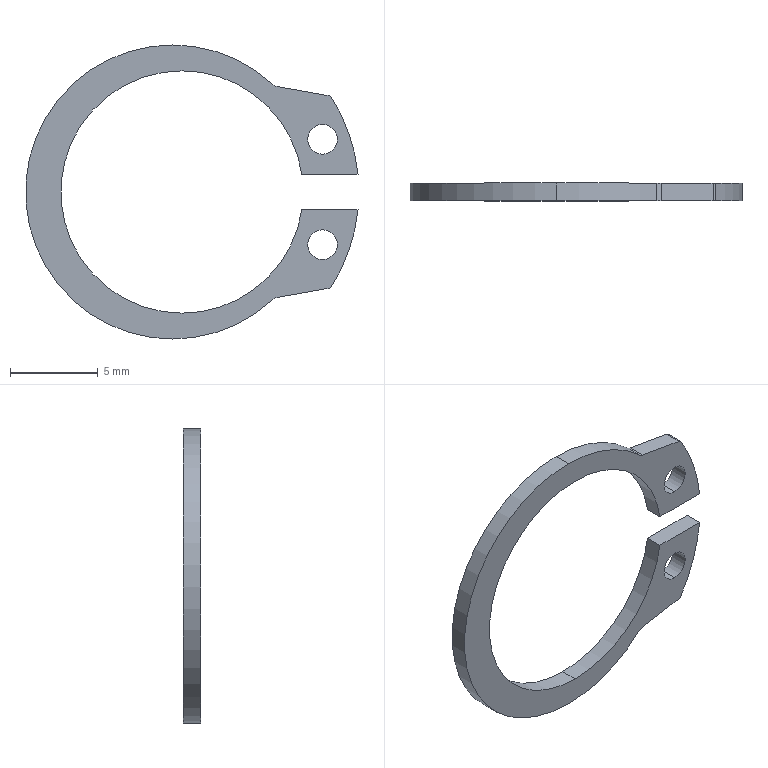Component | SolidWorks | 8TC-A15004-83-00-16_circlips for shaft--type a large gb-1 | 1 solid | 22 faces | volume 87 mm3 | cylinder 16 | plane 6 | commonest cylinder face diameters 1.7 x4 16.75 x3 13.8 x3 20.15 x2 0.4 x2 1 x2